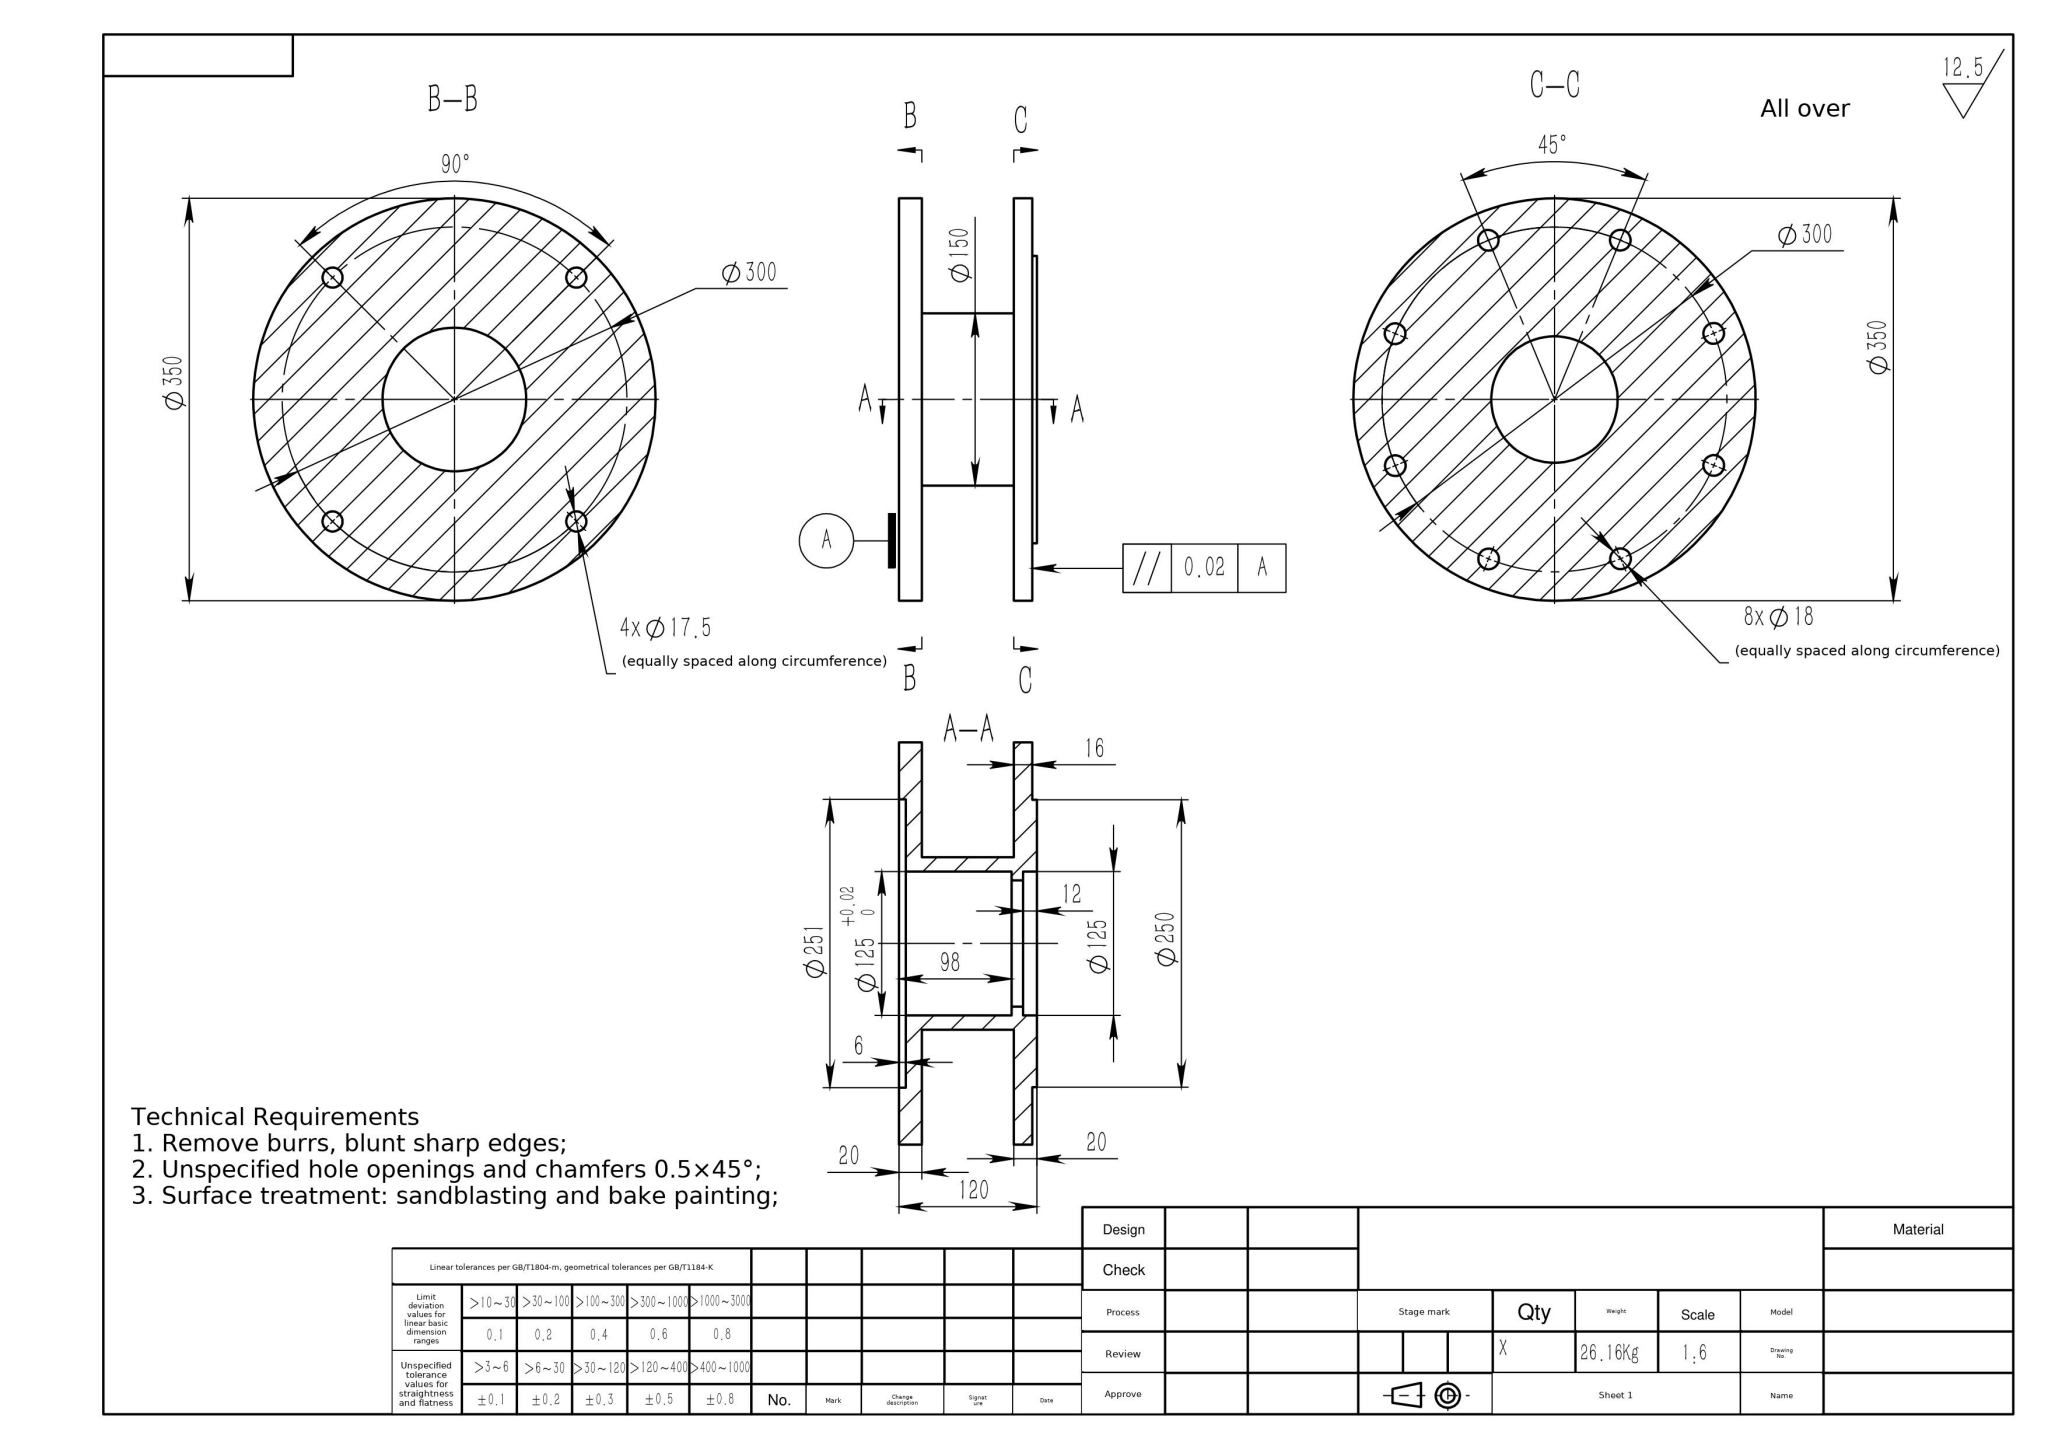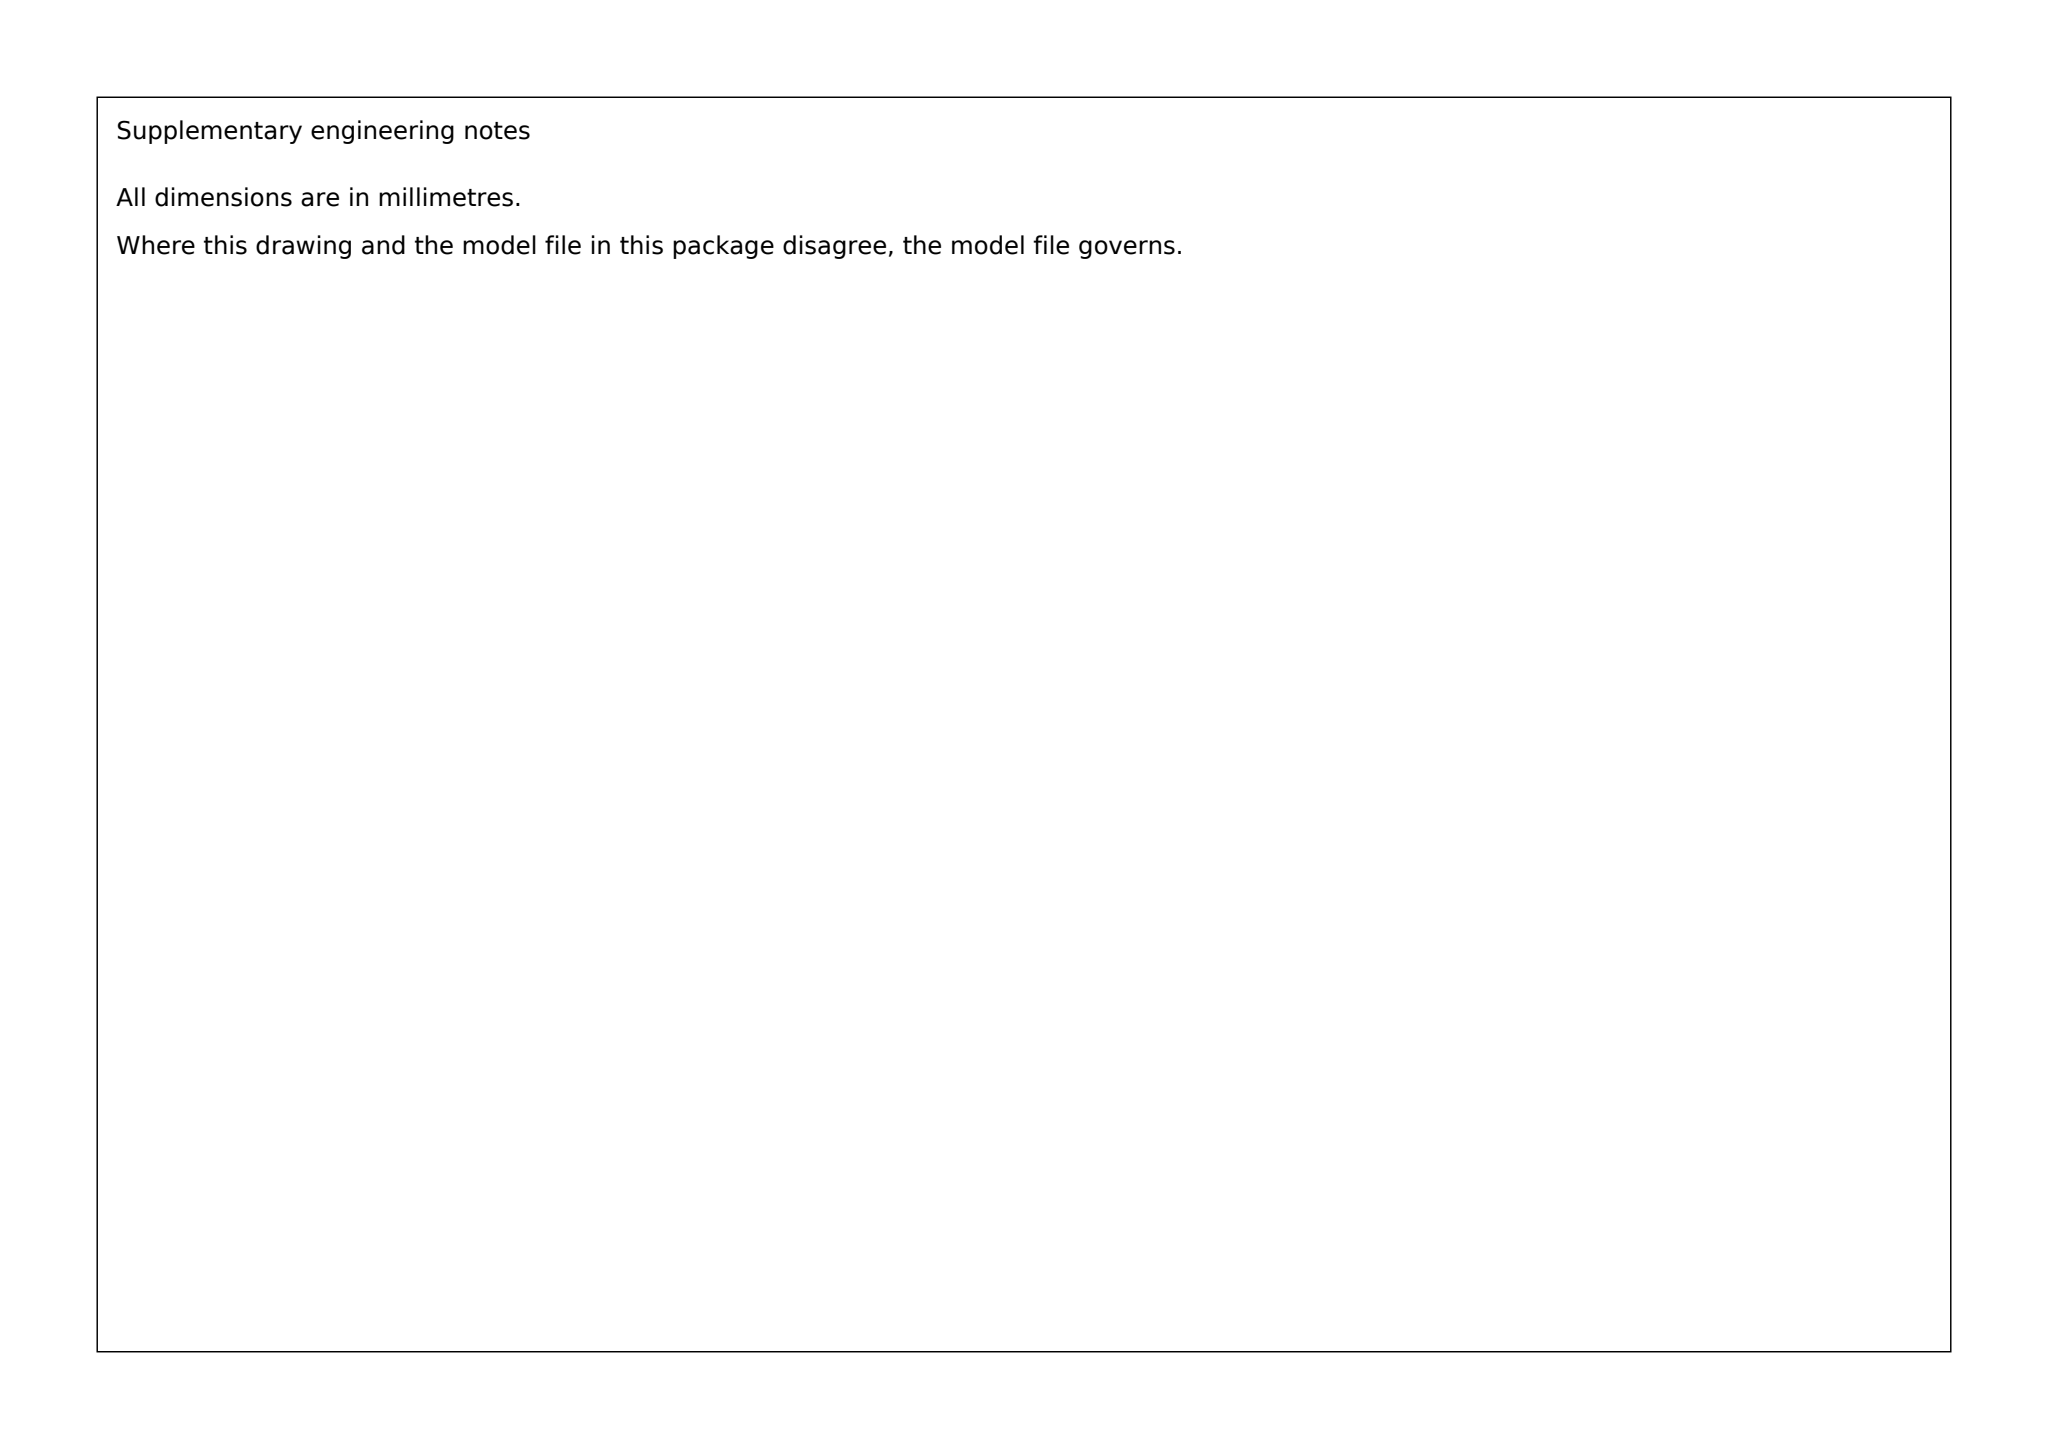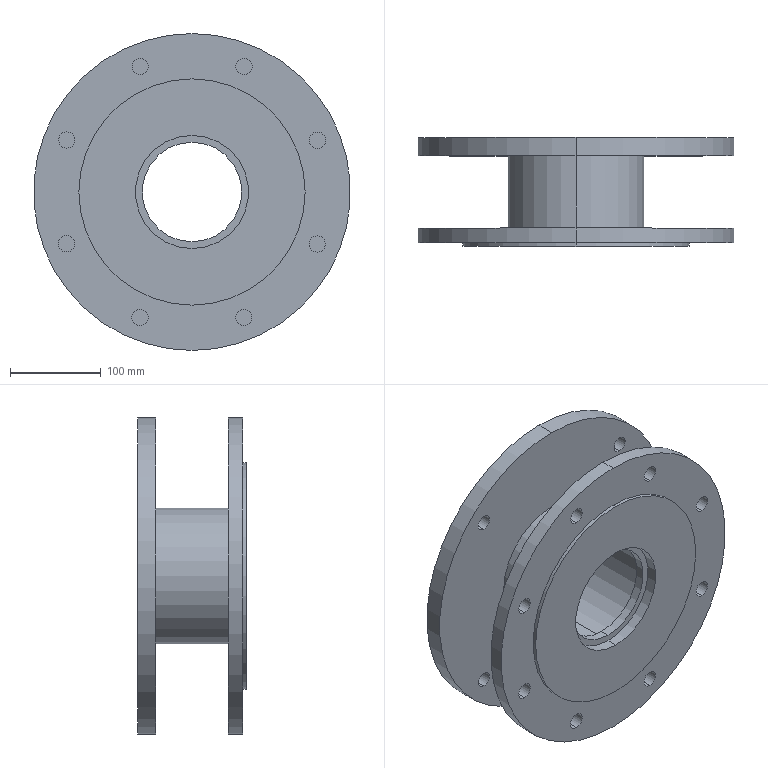Part | SolidWorks | mm | 1 solid | 48 faces | box 350 x 120 x 350 mm | volume 3353667 mm3 | cylinder 40 | plane 8 | commonest cylinder face diameters 18 x16 17.5 x8 125 x4 350 x4 250 x2 251 x2 110 x2 150 x2
build123d program:
from build123d import *

# Parameters (mm, degrees)
SKETCH2_R          = 125.5
CUT_EXTRUDE1_DEPTH = 6
CIRPATTERN1_COUNT  = 4
CIRPATTERN2_COUNT  = 8
SKETCH7_R          = 175
SKETCH7_R_2        = 125
CUT_EXTRUDE2_DEPTH = 4


with BuildPart() as part:
    # Sketch1 → Revolve1 (revolve)
    with BuildSketch(Plane.XY, mode=Mode.PRIVATE) as revolve1_sk:
        Polygon((62.5, 120), (175, 120), (175, 100), (75, 100), (75, 20), (175, 20), (175, 0), (62.5, 0), (62.5, 12), (55, 12), (55, 22), (62.5, 22), align=None)
    revolve(revolve1_sk.sketch.rotate(Axis((0, 0, 0), (0, 1, 0)), 90), axis=Axis((0, 0, 0), (0, 1, 0)))

    # Sketch2 → Cut-Extrude1 (cut)
    with BuildSketch(Plane(origin=(0, 120, 0), x_dir=(1, 0, 0), z_dir=(0, 1, 0))):
        with Locations(Location((0, 0, 0), (0, 0, 270))):
            Circle(SKETCH2_R)
    extrude(amount=-CUT_EXTRUDE1_DEPTH, mode=Mode.SUBTRACT)

    # Sketch4 → 17.5 _17.5_ Diameter Hole1 (revolve, cut)
    with BuildSketch(Plane(origin=(106.066, 120, -106.066), x_dir=(0, 0, 1), z_dir=(1, 0, 0))):
        Polygon((0, 0), (0, 44.508), (8.75, 39.25), (8.75, 0), align=None)
    f_17_5_17_5_diameter_hole1 = revolve(axis=Axis((106.066, 126.35, -106.066), (0, -1, 0)), mode=Mode.SUBTRACT)

    # CirPattern1: 17.5 _17.5_ Diameter Hole1 ×4 about axis
    cirpattern1_axis = Axis((0, 0, 0), (0, 1, 0))
    for i in range(1, CIRPATTERN1_COUNT):
        add(f_17_5_17_5_diameter_hole1.rotate(cirpattern1_axis, i * 360 / CIRPATTERN1_COUNT), mode=Mode.SUBTRACT)

    # Sketch6 → 18.0 _18_ Diameter Hole1 (revolve, cut)
    with BuildSketch(Plane(origin=(-138.532, 20, 57.523), x_dir=(0, 0, 1), z_dir=(1, 0, 0))):
        Polygon((0, 0), (0, 62.408), (9, 57), (9, 0), align=None)
    f_18_0_18_diameter_hole1 = revolve(axis=Axis((-138.532, 26.35, 57.523), (0, -1, 0)), mode=Mode.SUBTRACT)

    # CirPattern2: 18.0 _18_ Diameter Hole1 ×8 about axis
    cirpattern2_axis = Axis((0, 0, 0), (0, 1, 0))
    for i in range(1, CIRPATTERN2_COUNT):
        add(f_18_0_18_diameter_hole1.rotate(cirpattern2_axis, i * 360 / CIRPATTERN2_COUNT), mode=Mode.SUBTRACT)

    # Sketch7 → Cut-Extrude2 (cut)
    with BuildSketch(Plane.XZ):
        with Locations(Location((0, 0, 0), (0, 0, 270))):
            Circle(SKETCH7_R)
        with Locations(Location((0, 0, 0), (0, 0, 270))):
            Circle(SKETCH7_R_2, mode=Mode.SUBTRACT)
    extrude(amount=-CUT_EXTRUDE2_DEPTH, mode=Mode.SUBTRACT)


solid = part.part